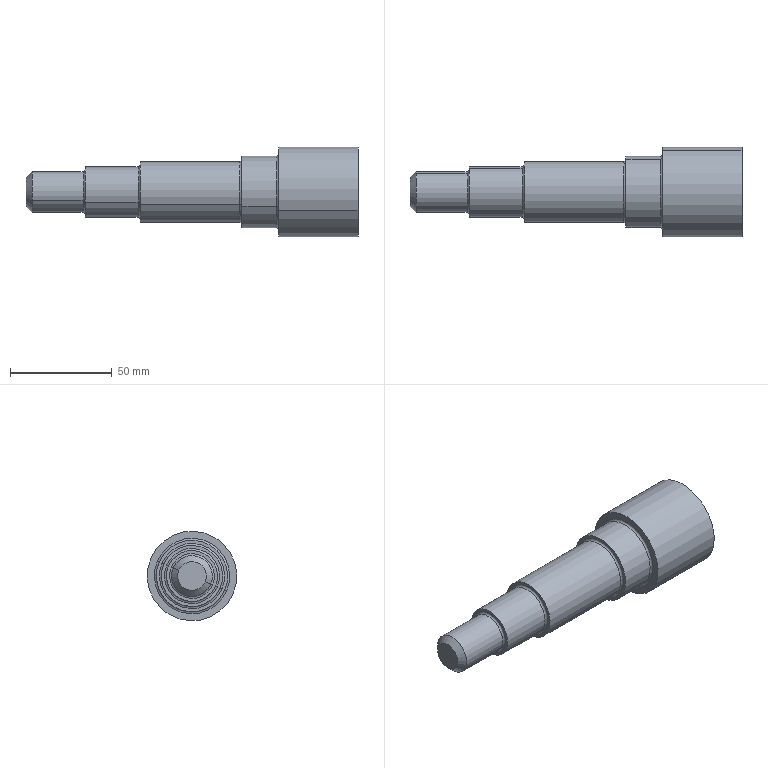Component | SolidWorks | AxisThree-1 | 1 solid | 26 faces | box 163 x 44 x 44 mm | volume 134147 mm3 | cylinder 10 | torus 8 | plane 6 | cone 2 | commonest cylinder face diameters 20 x2 25 x2 30 x2 35 x2 44 x2
build123d program:
from build123d import *


with BuildPart() as part:
    # Sketch1 → Revolve1 (revolve)
    with BuildSketch(Plane(origin=(0, 0, 0), x_dir=(0, 0, -1), z_dir=(1, 0, 0)), mode=Mode.PRIVATE) as revolve1_sk:
        with BuildLine():
            Line((0, 0), (0, 22))
            Line((0, 22), (39, 22))
            Line((39, 22), (39, 18.5))
            ThreePointArc((39, 18.5), (39.293, 17.793), (40, 17.5))
            Line((40, 17.5), (57, 17.5))
            Line((57, 17.5), (57, 16))
            ThreePointArc((57, 16), (57.293, 15.293), (58, 15))
            Line((58, 15), (107, 15))
            Line((107, 15), (107, 13.5))
            ThreePointArc((107, 13.5), (107.293, 12.793), (108, 12.5))
            Line((108, 12.5), (134, 12.5))
            Line((134, 12.5), (134, 11))
            ThreePointArc((134, 11), (134.293, 10.293), (135, 10))
            Line((135, 10), (160, 10))
            Line((160, 10), (163, 7))
            Line((163, 7), (163, 0))
            Line((163, 0), (0, 0))
        make_face()
    revolve(revolve1_sk.sketch.rotate(Axis((0, 0, -163), (0, 0, 1)), 90), axis=Axis((0, 0, -163), (0, 0, 1)))


solid = part.part

# Placed as in the assembly
solid = solid.moved(Location((528.528, 15.31, -240), (0, 90, 0)))
STEP:
#1=COLOUR_RGB('',0.7922,0.8196,0.9333);
#2=FILL_AREA_STYLE_COLOUR('',#1);
#3=FILL_AREA_STYLE('',(#2));
#4=SURFACE_STYLE_FILL_AREA(#3);
#5=SURFACE_SIDE_STYLE('',(#4));
#6=SURFACE_STYLE_USAGE(.BOTH.,#5);
#7=PRESENTATION_STYLE_ASSIGNMENT((#6));
#8=CARTESIAN_POINT('',(14.391,0.8549,-9.337));
#9=VERTEX_POINT('',#8);
#10=CARTESIAN_POINT('',(14.391,0.3507,-9.56));
#11=VERTEX_POINT('',#10);
#12=CARTESIAN_POINT('',(14.391,0.6028,-9.449));
#13=DIRECTION('',(-1.,0.,0.));
#14=DIRECTION('',(0.,0.9147,0.4041));
#15=AXIS2_PLACEMENT_3D('',#12,#13,#14);
#16=CIRCLE('',#15,0.2756);
#17=EDGE_CURVE('',#9,#11,#16,.T.);
#18=ORIENTED_EDGE('',*,*,#17,.F.);
#19=CARTESIAN_POINT('',(14.509,0.9629,-9.29));
#20=VERTEX_POINT('',#19);
#21=CARTESIAN_POINT('',(14.391,0.8549,-9.337));
#22=DIRECTION('',(0.7071,0.6468,0.2858));
#23=VECTOR('',#22,39.37);
#24=LINE('',#21,#23);
#25=EDGE_CURVE('',#9,#20,#24,.T.);
#26=ORIENTED_EDGE('',*,*,#25,.T.);
#27=CARTESIAN_POINT('',(14.509,0.2426,-9.608));
#28=VERTEX_POINT('',#27);
#29=CARTESIAN_POINT('',(14.509,0.6028,-9.449));
#30=DIRECTION('',(-1.,0.,0.));
#31=DIRECTION('',(0.,0.9147,0.4041));
#32=AXIS2_PLACEMENT_3D('',#29,#30,#31);
#33=CIRCLE('',#32,0.3937);
#34=EDGE_CURVE('',#20,#28,#33,.T.);
#35=ORIENTED_EDGE('',*,*,#34,.T.);
#36=CARTESIAN_POINT('',(14.391,0.3507,-9.56));
#37=DIRECTION('',(0.7071,-0.6468,-0.2858));
#38=VECTOR('',#37,39.37);
#39=LINE('',#36,#38);
#40=EDGE_CURVE('',#11,#28,#39,.T.);
#41=ORIENTED_EDGE('',*,*,#40,.F.);
#42=EDGE_LOOP('',(#18,#26,#35,#41));
#43=FACE_OUTER_BOUND('',#42,.T.);
#44=CARTESIAN_POINT('',(14.391,0.6028,-9.449));
#45=DIRECTION('',(1.,0.,0.));
#46=DIRECTION('',(0.,-0.9147,-0.4041));
#47=AXIS2_PLACEMENT_3D('',#44,#45,#46);
#48=CONICAL_SURFACE('',#47,0.2756,0.7854);
#49=ADVANCED_FACE('',(#43),#48,.T.);
#50=CARTESIAN_POINT('',(15.493,0.9629,-9.29));
#51=VERTEX_POINT('',#50);
#52=CARTESIAN_POINT('',(15.493,0.2426,-9.608));
#53=VERTEX_POINT('',#52);
#54=CARTESIAN_POINT('',(15.493,0.6028,-9.449));
#55=DIRECTION('',(-1.,0.,0.));
#56=DIRECTION('',(0.,0.9147,0.4041));
#57=AXIS2_PLACEMENT_3D('',#54,#55,#56);
#58=CIRCLE('',#57,0.3937);
#59=EDGE_CURVE('',#51,#53,#58,.T.);
#60=ORIENTED_EDGE('',*,*,#59,.T.);
#61=CARTESIAN_POINT('',(14.391,0.2426,-9.608));
#62=DIRECTION('',(-1.,0.,0.));
#63=VECTOR('',#62,39.37);
#64=LINE('',#61,#63);
#65=EDGE_CURVE('',#53,#28,#64,.T.);
#66=ORIENTED_EDGE('',*,*,#65,.T.);
#67=ORIENTED_EDGE('',*,*,#34,.F.);
#68=CARTESIAN_POINT('',(14.391,0.9629,-9.29));
#69=DIRECTION('',(-1.,0.,0.));
#70=VECTOR('',#69,39.37);
#71=LINE('',#68,#70);
#72=EDGE_CURVE('',#51,#20,#71,.T.);
#73=ORIENTED_EDGE('',*,*,#72,.F.);
#74=EDGE_LOOP('',(#60,#66,#67,#73));
#75=FACE_OUTER_BOUND('',#74,.T.);
#76=CARTESIAN_POINT('',(14.391,0.6028,-9.449));
#77=DIRECTION('',(-1.,0.,0.));
#78=DIRECTION('',(0.,0.9147,0.4041));
#79=AXIS2_PLACEMENT_3D('',#76,#77,#78);
#80=CYLINDRICAL_SURFACE('',#79,0.3937);
#81=ADVANCED_FACE('',(#75),#80,.T.);
#82=CARTESIAN_POINT('',(15.493,0.6028,-9.449));
#83=DIRECTION('',(-1.,0.,0.));
#84=DIRECTION('',(0.,0.9147,0.4041));
#85=AXIS2_PLACEMENT_3D('',#82,#83,#84);
#86=CIRCLE('',#85,0.3937);
#87=EDGE_CURVE('',#53,#51,#86,.T.);
#88=ORIENTED_EDGE('',*,*,#87,.F.);
#89=CARTESIAN_POINT('',(15.533,0.2066,-9.624));
#90=VERTEX_POINT('',#89);
#91=CARTESIAN_POINT('',(15.493,0.2066,-9.624));
#92=DIRECTION('',(0.,0.4041,-0.9147));
#93=DIRECTION('',(0.,0.9147,0.4041));
#94=AXIS2_PLACEMENT_3D('',#91,#92,#93);
#95=CIRCLE('',#94,0.03937);
#96=EDGE_CURVE('',#53,#90,#95,.T.);
#97=ORIENTED_EDGE('',*,*,#96,.T.);
#98=CARTESIAN_POINT('',(15.533,0.9989,-9.274));
#99=VERTEX_POINT('',#98);
#100=CARTESIAN_POINT('',(15.533,0.6028,-9.449));
#101=DIRECTION('',(-1.,0.,0.));
#102=DIRECTION('',(0.,0.9147,0.4041));
#103=AXIS2_PLACEMENT_3D('',#100,#101,#102);
#104=CIRCLE('',#103,0.4331);
#105=EDGE_CURVE('',#90,#99,#104,.T.);
#106=ORIENTED_EDGE('',*,*,#105,.T.);
#107=CARTESIAN_POINT('',(15.493,0.9989,-9.274));
#108=DIRECTION('',(0.,-0.4041,0.9147));
#109=DIRECTION('',(0.,-0.9147,-0.4041));
#110=AXIS2_PLACEMENT_3D('',#107,#108,#109);
#111=CIRCLE('',#110,0.03937);
#112=EDGE_CURVE('',#51,#99,#111,.T.);
#113=ORIENTED_EDGE('',*,*,#112,.F.);
#114=EDGE_LOOP('',(#88,#97,#106,#113));
#115=FACE_OUTER_BOUND('',#114,.T.);
#116=CARTESIAN_POINT('',(15.493,0.6028,-9.449));
#117=DIRECTION('',(-1.,0.,0.));
#118=DIRECTION('',(0.,0.9147,0.4041));
#119=AXIS2_PLACEMENT_3D('',#116,#117,#118);
#120=TOROIDAL_SURFACE('',#119,0.4331,0.03937);
#121=ADVANCED_FACE('',(#115),#120,.F.);
#122=CARTESIAN_POINT('',(16.556,1.053,-9.25));
#123=VERTEX_POINT('',#122);
#124=CARTESIAN_POINT('',(16.556,0.1526,-9.648));
#125=VERTEX_POINT('',#124);
#126=CARTESIAN_POINT('',(16.556,0.6028,-9.449));
#127=DIRECTION('',(-1.,0.,0.));
#128=DIRECTION('',(0.,0.9147,0.4041));
#129=AXIS2_PLACEMENT_3D('',#126,#127,#128);
#130=CIRCLE('',#129,0.4921);
#131=EDGE_CURVE('',#123,#125,#130,.T.);
#132=ORIENTED_EDGE('',*,*,#131,.T.);
#133=CARTESIAN_POINT('',(15.533,0.1526,-9.648));
#134=VERTEX_POINT('',#133);
#135=CARTESIAN_POINT('',(14.391,0.1526,-9.648));
#136=DIRECTION('',(-1.,0.,0.));
#137=VECTOR('',#136,39.37);
#138=LINE('',#135,#137);
#139=EDGE_CURVE('',#125,#134,#138,.T.);
#140=ORIENTED_EDGE('',*,*,#139,.T.);
#141=CARTESIAN_POINT('',(15.533,1.053,-9.25));
#142=VERTEX_POINT('',#141);
#143=CARTESIAN_POINT('',(15.533,0.6028,-9.449));
#144=DIRECTION('',(-1.,0.,0.));
#145=DIRECTION('',(0.,0.9147,0.4041));
#146=AXIS2_PLACEMENT_3D('',#143,#144,#145);
#147=CIRCLE('',#146,0.4921);
#148=EDGE_CURVE('',#142,#134,#147,.T.);
#149=ORIENTED_EDGE('',*,*,#148,.F.);
#150=CARTESIAN_POINT('',(14.391,1.053,-9.25));
#151=DIRECTION('',(-1.,0.,0.));
#152=VECTOR('',#151,39.37);
#153=LINE('',#150,#152);
#154=EDGE_CURVE('',#123,#142,#153,.T.);
#155=ORIENTED_EDGE('',*,*,#154,.F.);
#156=EDGE_LOOP('',(#132,#140,#149,#155));
#157=FACE_OUTER_BOUND('',#156,.T.);
#158=CARTESIAN_POINT('',(14.391,0.6028,-9.449));
#159=DIRECTION('',(-1.,0.,0.));
#160=DIRECTION('',(0.,0.9147,0.4041));
#161=AXIS2_PLACEMENT_3D('',#158,#159,#160);
#162=CYLINDRICAL_SURFACE('',#161,0.4921);
#163=ADVANCED_FACE('',(#157),#162,.T.);
#164=CARTESIAN_POINT('',(16.556,0.6028,-9.449));
#165=DIRECTION('',(-1.,0.,0.));
#166=DIRECTION('',(0.,0.9147,0.4041));
#167=AXIS2_PLACEMENT_3D('',#164,#165,#166);
#168=CIRCLE('',#167,0.4921);
#169=EDGE_CURVE('',#125,#123,#168,.T.);
#170=ORIENTED_EDGE('',*,*,#169,.F.);
#171=CARTESIAN_POINT('',(16.596,0.1166,-9.664));
#172=VERTEX_POINT('',#171);
#173=CARTESIAN_POINT('',(16.556,0.1166,-9.664));
#174=DIRECTION('',(0.,0.4041,-0.9147));
#175=DIRECTION('',(0.,0.9147,0.4041));
#176=AXIS2_PLACEMENT_3D('',#173,#174,#175);
#177=CIRCLE('',#176,0.03937);
#178=EDGE_CURVE('',#125,#172,#177,.T.);
#179=ORIENTED_EDGE('',*,*,#178,.T.);
#180=CARTESIAN_POINT('',(16.596,1.089,-9.234));
#181=VERTEX_POINT('',#180);
#182=CARTESIAN_POINT('',(16.596,0.6028,-9.449));
#183=DIRECTION('',(-1.,0.,0.));
#184=DIRECTION('',(0.,0.9147,0.4041));
#185=AXIS2_PLACEMENT_3D('',#182,#183,#184);
#186=CIRCLE('',#185,0.5315);
#187=EDGE_CURVE('',#172,#181,#186,.T.);
#188=ORIENTED_EDGE('',*,*,#187,.T.);
#189=CARTESIAN_POINT('',(16.556,1.089,-9.234));
#190=DIRECTION('',(0.,-0.4041,0.9147));
#191=DIRECTION('',(0.,-0.9147,-0.4041));
#192=AXIS2_PLACEMENT_3D('',#189,#190,#191);
#193=CIRCLE('',#192,0.03937);
#194=EDGE_CURVE('',#123,#181,#193,.T.);
#195=ORIENTED_EDGE('',*,*,#194,.F.);
#196=EDGE_LOOP('',(#170,#179,#188,#195));
#197=FACE_OUTER_BOUND('',#196,.T.);
#198=CARTESIAN_POINT('',(16.556,0.6028,-9.449));
#199=DIRECTION('',(-1.,0.,0.));
#200=DIRECTION('',(0.,0.9147,0.4041));
#201=AXIS2_PLACEMENT_3D('',#198,#199,#200);
#202=TOROIDAL_SURFACE('',#201,0.5315,0.03937);
#203=ADVANCED_FACE('',(#197),#202,.F.);
#204=CARTESIAN_POINT('',(18.525,1.143,-9.21));
#205=VERTEX_POINT('',#204);
#206=CARTESIAN_POINT('',(18.525,0.06259,-9.687));
#207=VERTEX_POINT('',#206);
#208=CARTESIAN_POINT('',(18.525,0.6028,-9.449));
#209=DIRECTION('',(-1.,0.,0.));
#210=DIRECTION('',(0.,0.9147,0.4041));
#211=AXIS2_PLACEMENT_3D('',#208,#209,#210);
#212=CIRCLE('',#211,0.5906);
#213=EDGE_CURVE('',#205,#207,#212,.T.);
#214=ORIENTED_EDGE('',*,*,#213,.T.);
#215=CARTESIAN_POINT('',(16.596,0.06259,-9.687));
#216=VERTEX_POINT('',#215);
#217=CARTESIAN_POINT('',(14.391,0.06259,-9.687));
#218=DIRECTION('',(-1.,0.,0.));
#219=VECTOR('',#218,39.37);
#220=LINE('',#217,#219);
#221=EDGE_CURVE('',#207,#216,#220,.T.);
#222=ORIENTED_EDGE('',*,*,#221,.T.);
#223=CARTESIAN_POINT('',(16.596,1.143,-9.21));
#224=VERTEX_POINT('',#223);
#225=CARTESIAN_POINT('',(16.596,0.6028,-9.449));
#226=DIRECTION('',(-1.,0.,0.));
#227=DIRECTION('',(0.,0.9147,0.4041));
#228=AXIS2_PLACEMENT_3D('',#225,#226,#227);
#229=CIRCLE('',#228,0.5906);
#230=EDGE_CURVE('',#224,#216,#229,.T.);
#231=ORIENTED_EDGE('',*,*,#230,.F.);
#232=CARTESIAN_POINT('',(14.391,1.143,-9.21));
#233=DIRECTION('',(-1.,0.,0.));
#234=VECTOR('',#233,39.37);
#235=LINE('',#232,#234);
#236=EDGE_CURVE('',#205,#224,#235,.T.);
#237=ORIENTED_EDGE('',*,*,#236,.F.);
#238=EDGE_LOOP('',(#214,#222,#231,#237));
#239=FACE_OUTER_BOUND('',#238,.T.);
#240=CARTESIAN_POINT('',(14.391,0.6028,-9.449));
#241=DIRECTION('',(-1.,0.,0.));
#242=DIRECTION('',(0.,0.9147,0.4041));
#243=AXIS2_PLACEMENT_3D('',#240,#241,#242);
#244=CYLINDRICAL_SURFACE('',#243,0.5906);
#245=ADVANCED_FACE('',(#239),#244,.T.);
#246=CARTESIAN_POINT('',(18.525,0.6028,-9.449));
#247=DIRECTION('',(-1.,0.,0.));
#248=DIRECTION('',(0.,0.9147,0.4041));
#249=AXIS2_PLACEMENT_3D('',#246,#247,#248);
#250=CIRCLE('',#249,0.5906);
#251=EDGE_CURVE('',#207,#205,#250,.T.);
#252=ORIENTED_EDGE('',*,*,#251,.F.);
#253=CARTESIAN_POINT('',(18.564,0.02658,-9.703));
#254=VERTEX_POINT('',#253);
#255=CARTESIAN_POINT('',(18.525,0.02658,-9.703));
#256=DIRECTION('',(0.,0.4041,-0.9147));
#257=DIRECTION('',(0.,0.9147,0.4041));
#258=AXIS2_PLACEMENT_3D('',#255,#256,#257);
#259=CIRCLE('',#258,0.03937);
#260=EDGE_CURVE('',#207,#254,#259,.T.);
#261=ORIENTED_EDGE('',*,*,#260,.T.);
#262=CARTESIAN_POINT('',(18.564,1.179,-9.194));
#263=VERTEX_POINT('',#262);
#264=CARTESIAN_POINT('',(18.564,0.6028,-9.449));
#265=DIRECTION('',(-1.,0.,0.));
#266=DIRECTION('',(0.,0.9147,0.4041));
#267=AXIS2_PLACEMENT_3D('',#264,#265,#266);
#268=CIRCLE('',#267,0.6299);
#269=EDGE_CURVE('',#254,#263,#268,.T.);
#270=ORIENTED_EDGE('',*,*,#269,.T.);
#271=CARTESIAN_POINT('',(18.525,1.179,-9.194));
#272=DIRECTION('',(0.,-0.4041,0.9147));
#273=DIRECTION('',(0.,-0.9147,-0.4041));
#274=AXIS2_PLACEMENT_3D('',#271,#272,#273);
#275=CIRCLE('',#274,0.03937);
#276=EDGE_CURVE('',#205,#263,#275,.T.);
#277=ORIENTED_EDGE('',*,*,#276,.F.);
#278=EDGE_LOOP('',(#252,#261,#270,#277));
#279=FACE_OUTER_BOUND('',#278,.T.);
#280=CARTESIAN_POINT('',(18.525,0.6028,-9.449));
#281=DIRECTION('',(-1.,0.,0.));
#282=DIRECTION('',(0.,0.9147,0.4041));
#283=AXIS2_PLACEMENT_3D('',#280,#281,#282);
#284=TOROIDAL_SURFACE('',#283,0.6299,0.03937);
#285=ADVANCED_FACE('',(#279),#284,.F.);
#286=CARTESIAN_POINT('',(19.233,1.233,-9.17));
#287=VERTEX_POINT('',#286);
#288=CARTESIAN_POINT('',(19.233,-0.02744,-9.727));
#289=VERTEX_POINT('',#288);
#290=CARTESIAN_POINT('',(19.233,0.6028,-9.449));
#291=DIRECTION('',(-1.,0.,0.));
#292=DIRECTION('',(0.,0.9147,0.4041));
#293=AXIS2_PLACEMENT_3D('',#290,#291,#292);
#294=CIRCLE('',#293,0.689);
#295=EDGE_CURVE('',#287,#289,#294,.T.);
#296=ORIENTED_EDGE('',*,*,#295,.T.);
#297=CARTESIAN_POINT('',(18.564,-0.02744,-9.727));
#298=VERTEX_POINT('',#297);
#299=CARTESIAN_POINT('',(14.391,-0.02744,-9.727));
#300=DIRECTION('',(-1.,0.,0.));
#301=VECTOR('',#300,39.37);
#302=LINE('',#299,#301);
#303=EDGE_CURVE('',#289,#298,#302,.T.);
#304=ORIENTED_EDGE('',*,*,#303,.T.);
#305=CARTESIAN_POINT('',(18.564,1.233,-9.17));
#306=VERTEX_POINT('',#305);
#307=CARTESIAN_POINT('',(18.564,0.6028,-9.449));
#308=DIRECTION('',(-1.,0.,0.));
#309=DIRECTION('',(0.,0.9147,0.4041));
#310=AXIS2_PLACEMENT_3D('',#307,#308,#309);
#311=CIRCLE('',#310,0.689);
#312=EDGE_CURVE('',#306,#298,#311,.T.);
#313=ORIENTED_EDGE('',*,*,#312,.F.);
#314=CARTESIAN_POINT('',(14.391,1.233,-9.17));
#315=DIRECTION('',(-1.,0.,0.));
#316=VECTOR('',#315,39.37);
#317=LINE('',#314,#316);
#318=EDGE_CURVE('',#287,#306,#317,.T.);
#319=ORIENTED_EDGE('',*,*,#318,.F.);
#320=EDGE_LOOP('',(#296,#304,#313,#319));
#321=FACE_OUTER_BOUND('',#320,.T.);
#322=CARTESIAN_POINT('',(14.391,0.6028,-9.449));
#323=DIRECTION('',(-1.,0.,0.));
#324=DIRECTION('',(0.,0.9147,0.4041));
#325=AXIS2_PLACEMENT_3D('',#322,#323,#324);
#326=CYLINDRICAL_SURFACE('',#325,0.689);
#327=ADVANCED_FACE('',(#321),#326,.T.);
#328=CARTESIAN_POINT('',(19.233,0.6028,-9.449));
#329=DIRECTION('',(-1.,0.,0.));
#330=DIRECTION('',(0.,0.9147,0.4041));
#331=AXIS2_PLACEMENT_3D('',#328,#329,#330);
#332=CIRCLE('',#331,0.689);
#333=EDGE_CURVE('',#289,#287,#332,.T.);
#334=ORIENTED_EDGE('',*,*,#333,.F.);
#335=CARTESIAN_POINT('',(19.273,-0.06345,-9.743));
#336=VERTEX_POINT('',#335);
#337=CARTESIAN_POINT('',(19.233,-0.06345,-9.743));
#338=DIRECTION('',(0.,0.4041,-0.9147));
#339=DIRECTION('',(0.,0.9147,0.4041));
#340=AXIS2_PLACEMENT_3D('',#337,#338,#339);
#341=CIRCLE('',#340,0.03937);
#342=EDGE_CURVE('',#289,#336,#341,.T.);
#343=ORIENTED_EDGE('',*,*,#342,.T.);
#344=CARTESIAN_POINT('',(19.273,1.269,-9.154));
#345=VERTEX_POINT('',#344);
#346=CARTESIAN_POINT('',(19.273,0.6028,-9.449));
#347=DIRECTION('',(-1.,0.,0.));
#348=DIRECTION('',(0.,0.9147,0.4041));
#349=AXIS2_PLACEMENT_3D('',#346,#347,#348);
#350=CIRCLE('',#349,0.7283);
#351=EDGE_CURVE('',#336,#345,#350,.T.);
#352=ORIENTED_EDGE('',*,*,#351,.T.);
#353=CARTESIAN_POINT('',(19.233,1.269,-9.154));
#354=DIRECTION('',(0.,-0.4041,0.9147));
#355=DIRECTION('',(0.,-0.9147,-0.4041));
#356=AXIS2_PLACEMENT_3D('',#353,#354,#355);
#357=CIRCLE('',#356,0.03937);
#358=EDGE_CURVE('',#287,#345,#357,.T.);
#359=ORIENTED_EDGE('',*,*,#358,.F.);
#360=EDGE_LOOP('',(#334,#343,#352,#359));
#361=FACE_OUTER_BOUND('',#360,.T.);
#362=CARTESIAN_POINT('',(19.233,0.6028,-9.449));
#363=DIRECTION('',(-1.,0.,0.));
#364=DIRECTION('',(0.,0.9147,0.4041));
#365=AXIS2_PLACEMENT_3D('',#362,#363,#364);
#366=TOROIDAL_SURFACE('',#365,0.7283,0.03937);
#367=ADVANCED_FACE('',(#361),#366,.F.);
#368=CARTESIAN_POINT('',(20.808,1.395,-9.099));
#369=VERTEX_POINT('',#368);
#370=CARTESIAN_POINT('',(20.808,-0.1895,-9.799));
#371=VERTEX_POINT('',#370);
#372=CARTESIAN_POINT('',(20.808,0.6028,-9.449));
#373=DIRECTION('',(-1.,0.,0.));
#374=DIRECTION('',(0.,0.9147,0.4041));
#375=AXIS2_PLACEMENT_3D('',#372,#373,#374);
#376=CIRCLE('',#375,0.8661);
#377=EDGE_CURVE('',#369,#371,#376,.T.);
#378=ORIENTED_EDGE('',*,*,#377,.T.);
#379=CARTESIAN_POINT('',(19.273,-0.1895,-9.799));
#380=VERTEX_POINT('',#379);
#381=CARTESIAN_POINT('',(14.391,-0.1895,-9.799));
#382=DIRECTION('',(-1.,0.,0.));
#383=VECTOR('',#382,39.37);
#384=LINE('',#381,#383);
#385=EDGE_CURVE('',#371,#380,#384,.T.);
#386=ORIENTED_EDGE('',*,*,#385,.T.);
#387=CARTESIAN_POINT('',(19.273,1.395,-9.099));
#388=VERTEX_POINT('',#387);
#389=CARTESIAN_POINT('',(19.273,0.6028,-9.449));
#390=DIRECTION('',(-1.,0.,0.));
#391=DIRECTION('',(0.,0.9147,0.4041));
#392=AXIS2_PLACEMENT_3D('',#389,#390,#391);
#393=CIRCLE('',#392,0.8661);
#394=EDGE_CURVE('',#388,#380,#393,.T.);
#395=ORIENTED_EDGE('',*,*,#394,.F.);
#396=CARTESIAN_POINT('',(14.391,1.395,-9.099));
#397=DIRECTION('',(-1.,0.,0.));
#398=VECTOR('',#397,39.37);
#399=LINE('',#396,#398);
#400=EDGE_CURVE('',#369,#388,#399,.T.);
#401=ORIENTED_EDGE('',*,*,#400,.F.);
#402=EDGE_LOOP('',(#378,#386,#395,#401));
#403=FACE_OUTER_BOUND('',#402,.T.);
#404=CARTESIAN_POINT('',(14.391,0.6028,-9.449));
#405=DIRECTION('',(-1.,0.,0.));
#406=DIRECTION('',(0.,0.9147,0.4041));
#407=AXIS2_PLACEMENT_3D('',#404,#405,#406);
#408=CYLINDRICAL_SURFACE('',#407,0.8661);
#409=ADVANCED_FACE('',(#403),#408,.T.);
#410=ORIENTED_EDGE('',*,*,#377,.F.);
#411=CARTESIAN_POINT('',(20.808,0.6028,-9.449));
#412=DIRECTION('',(-1.,0.,0.));
#413=DIRECTION('',(0.,0.9147,0.4041));
#414=AXIS2_PLACEMENT_3D('',#411,#412,#413);
#415=CIRCLE('',#414,0.8661);
#416=EDGE_CURVE('',#371,#369,#415,.T.);
#417=ORIENTED_EDGE('',*,*,#416,.F.);
#418=EDGE_LOOP('',(#410,#417));
#419=FACE_OUTER_BOUND('',#418,.T.);
#420=CARTESIAN_POINT('',(20.808,0.6028,-9.449));
#421=DIRECTION('',(1.,0.,0.));
#422=DIRECTION('',(0.,-0.9147,-0.4041));
#423=AXIS2_PLACEMENT_3D('',#420,#421,#422);
#424=PLANE('',#423);
#425=ADVANCED_FACE('',(#419),#424,.T.);
#426=ORIENTED_EDGE('',*,*,#385,.F.);
#427=ORIENTED_EDGE('',*,*,#416,.T.);
#428=ORIENTED_EDGE('',*,*,#400,.T.);
#429=CARTESIAN_POINT('',(19.273,0.6028,-9.449));
#430=DIRECTION('',(-1.,0.,0.));
#431=DIRECTION('',(0.,0.9147,0.4041));
#432=AXIS2_PLACEMENT_3D('',#429,#430,#431);
#433=CIRCLE('',#432,0.8661);
#434=EDGE_CURVE('',#380,#388,#433,.T.);
#435=ORIENTED_EDGE('',*,*,#434,.F.);
#436=EDGE_LOOP('',(#426,#427,#428,#435));
#437=FACE_OUTER_BOUND('',#436,.T.);
#438=CARTESIAN_POINT('',(14.391,0.6028,-9.449));
#439=DIRECTION('',(-1.,0.,0.));
#440=DIRECTION('',(0.,0.9147,0.4041));
#441=AXIS2_PLACEMENT_3D('',#438,#439,#440);
#442=CYLINDRICAL_SURFACE('',#441,0.8661);
#443=ADVANCED_FACE('',(#437),#442,.T.);
#444=ORIENTED_EDGE('',*,*,#394,.T.);
#445=ORIENTED_EDGE('',*,*,#434,.T.);
#446=EDGE_LOOP('',(#444,#445));
#447=FACE_OUTER_BOUND('',#446,.T.);
#448=CARTESIAN_POINT('',(19.273,0.6028,-9.449));
#449=DIRECTION('',(-1.,0.,0.));
#450=DIRECTION('',(0.,0.9147,0.4041));
#451=AXIS2_PLACEMENT_3D('',#448,#449,#450);
#452=CIRCLE('',#451,0.7283);
#453=EDGE_CURVE('',#345,#336,#452,.T.);
#454=ORIENTED_EDGE('',*,*,#453,.F.);
#455=ORIENTED_EDGE('',*,*,#351,.F.);
#456=EDGE_LOOP('',(#454,#455));
#457=FACE_BOUND('',#456,.T.);
#458=CARTESIAN_POINT('',(19.273,0.9528,-10.241));
#459=DIRECTION('',(-1.,0.,0.));
#460=DIRECTION('',(0.,0.9147,0.4041));
#461=AXIS2_PLACEMENT_3D('',#458,#459,#460);
#462=PLANE('',#461);
#463=ADVANCED_FACE('',(#447,#457),#462,.T.);
#464=ORIENTED_EDGE('',*,*,#342,.F.);
#465=ORIENTED_EDGE('',*,*,#295,.F.);
#466=ORIENTED_EDGE('',*,*,#358,.T.);
#467=ORIENTED_EDGE('',*,*,#453,.T.);
#468=EDGE_LOOP('',(#464,#465,#466,#467));
#469=FACE_OUTER_BOUND('',#468,.T.);
#470=CARTESIAN_POINT('',(19.233,0.6028,-9.449));
#471=DIRECTION('',(-1.,0.,0.));
#472=DIRECTION('',(0.,0.9147,0.4041));
#473=AXIS2_PLACEMENT_3D('',#470,#471,#472);
#474=TOROIDAL_SURFACE('',#473,0.7283,0.03937);
#475=ADVANCED_FACE('',(#469),#474,.F.);
#476=ORIENTED_EDGE('',*,*,#303,.F.);
#477=ORIENTED_EDGE('',*,*,#333,.T.);
#478=ORIENTED_EDGE('',*,*,#318,.T.);
#479=CARTESIAN_POINT('',(18.564,0.6028,-9.449));
#480=DIRECTION('',(-1.,0.,0.));
#481=DIRECTION('',(0.,0.9147,0.4041));
#482=AXIS2_PLACEMENT_3D('',#479,#480,#481);
#483=CIRCLE('',#482,0.689);
#484=EDGE_CURVE('',#298,#306,#483,.T.);
#485=ORIENTED_EDGE('',*,*,#484,.F.);
#486=EDGE_LOOP('',(#476,#477,#478,#485));
#487=FACE_OUTER_BOUND('',#486,.T.);
#488=CARTESIAN_POINT('',(14.391,0.6028,-9.449));
#489=DIRECTION('',(-1.,0.,0.));
#490=DIRECTION('',(0.,0.9147,0.4041));
#491=AXIS2_PLACEMENT_3D('',#488,#489,#490);
#492=CYLINDRICAL_SURFACE('',#491,0.689);
#493=ADVANCED_FACE('',(#487),#492,.T.);
#494=ORIENTED_EDGE('',*,*,#312,.T.);
#495=ORIENTED_EDGE('',*,*,#484,.T.);
#496=EDGE_LOOP('',(#494,#495));
#497=FACE_OUTER_BOUND('',#496,.T.);
#498=CARTESIAN_POINT('',(18.564,0.6028,-9.449));
#499=DIRECTION('',(-1.,0.,0.));
#500=DIRECTION('',(0.,0.9147,0.4041));
#501=AXIS2_PLACEMENT_3D('',#498,#499,#500);
#502=CIRCLE('',#501,0.6299);
#503=EDGE_CURVE('',#263,#254,#502,.T.);
#504=ORIENTED_EDGE('',*,*,#503,.F.);
#505=ORIENTED_EDGE('',*,*,#269,.F.);
#506=EDGE_LOOP('',(#504,#505));
#507=FACE_BOUND('',#506,.T.);
#508=CARTESIAN_POINT('',(18.564,0.8812,-10.079));
#509=DIRECTION('',(-1.,0.,0.));
#510=DIRECTION('',(0.,0.9147,0.4041));
#511=AXIS2_PLACEMENT_3D('',#508,#509,#510);
#512=PLANE('',#511);
#513=ADVANCED_FACE('',(#497,#507),#512,.T.);
#514=ORIENTED_EDGE('',*,*,#260,.F.);
#515=ORIENTED_EDGE('',*,*,#213,.F.);
#516=ORIENTED_EDGE('',*,*,#276,.T.);
#517=ORIENTED_EDGE('',*,*,#503,.T.);
#518=EDGE_LOOP('',(#514,#515,#516,#517));
#519=FACE_OUTER_BOUND('',#518,.T.);
#520=CARTESIAN_POINT('',(18.525,0.6028,-9.449));
#521=DIRECTION('',(-1.,0.,0.));
#522=DIRECTION('',(0.,0.9147,0.4041));
#523=AXIS2_PLACEMENT_3D('',#520,#521,#522);
#524=TOROIDAL_SURFACE('',#523,0.6299,0.03937);
#525=ADVANCED_FACE('',(#519),#524,.F.);
#526=ORIENTED_EDGE('',*,*,#221,.F.);
#527=ORIENTED_EDGE('',*,*,#251,.T.);
#528=ORIENTED_EDGE('',*,*,#236,.T.);
#529=CARTESIAN_POINT('',(16.596,0.6028,-9.449));
#530=DIRECTION('',(-1.,0.,0.));
#531=DIRECTION('',(0.,0.9147,0.4041));
#532=AXIS2_PLACEMENT_3D('',#529,#530,#531);
#533=CIRCLE('',#532,0.5906);
#534=EDGE_CURVE('',#216,#224,#533,.T.);
#535=ORIENTED_EDGE('',*,*,#534,.F.);
#536=EDGE_LOOP('',(#526,#527,#528,#535));
#537=FACE_OUTER_BOUND('',#536,.T.);
#538=CARTESIAN_POINT('',(14.391,0.6028,-9.449));
#539=DIRECTION('',(-1.,0.,0.));
#540=DIRECTION('',(0.,0.9147,0.4041));
#541=AXIS2_PLACEMENT_3D('',#538,#539,#540);
#542=CYLINDRICAL_SURFACE('',#541,0.5906);
#543=ADVANCED_FACE('',(#537),#542,.T.);
#544=ORIENTED_EDGE('',*,*,#230,.T.);
#545=ORIENTED_EDGE('',*,*,#534,.T.);
#546=EDGE_LOOP('',(#544,#545));
#547=FACE_OUTER_BOUND('',#546,.T.);
#548=CARTESIAN_POINT('',(16.596,0.6028,-9.449));
#549=DIRECTION('',(-1.,0.,0.));
#550=DIRECTION('',(0.,0.9147,0.4041));
#551=AXIS2_PLACEMENT_3D('',#548,#549,#550);
#552=CIRCLE('',#551,0.5315);
#553=EDGE_CURVE('',#181,#172,#552,.T.);
#554=ORIENTED_EDGE('',*,*,#553,.F.);
#555=ORIENTED_EDGE('',*,*,#187,.F.);
#556=EDGE_LOOP('',(#554,#555));
#557=FACE_BOUND('',#556,.T.);
#558=CARTESIAN_POINT('',(16.596,0.8414,-9.989));
#559=DIRECTION('',(-1.,0.,0.));
#560=DIRECTION('',(0.,0.9147,0.4041));
#561=AXIS2_PLACEMENT_3D('',#558,#559,#560);
#562=PLANE('',#561);
#563=ADVANCED_FACE('',(#547,#557),#562,.T.);
#564=ORIENTED_EDGE('',*,*,#178,.F.);
#565=ORIENTED_EDGE('',*,*,#131,.F.);
#566=ORIENTED_EDGE('',*,*,#194,.T.);
#567=ORIENTED_EDGE('',*,*,#553,.T.);
#568=EDGE_LOOP('',(#564,#565,#566,#567));
#569=FACE_OUTER_BOUND('',#568,.T.);
#570=CARTESIAN_POINT('',(16.556,0.6028,-9.449));
#571=DIRECTION('',(-1.,0.,0.));
#572=DIRECTION('',(0.,0.9147,0.4041));
#573=AXIS2_PLACEMENT_3D('',#570,#571,#572);
#574=TOROIDAL_SURFACE('',#573,0.5315,0.03937);
#575=ADVANCED_FACE('',(#569),#574,.F.);
#576=ORIENTED_EDGE('',*,*,#139,.F.);
#577=ORIENTED_EDGE('',*,*,#169,.T.);
#578=ORIENTED_EDGE('',*,*,#154,.T.);
#579=CARTESIAN_POINT('',(15.533,0.6028,-9.449));
#580=DIRECTION('',(-1.,0.,0.));
#581=DIRECTION('',(0.,0.9147,0.4041));
#582=AXIS2_PLACEMENT_3D('',#579,#580,#581);
#583=CIRCLE('',#582,0.4921);
#584=EDGE_CURVE('',#134,#142,#583,.T.);
#585=ORIENTED_EDGE('',*,*,#584,.F.);
#586=EDGE_LOOP('',(#576,#577,#578,#585));
#587=FACE_OUTER_BOUND('',#586,.T.);
#588=CARTESIAN_POINT('',(14.391,0.6028,-9.449));
#589=DIRECTION('',(-1.,0.,0.));
#590=DIRECTION('',(0.,0.9147,0.4041));
#591=AXIS2_PLACEMENT_3D('',#588,#589,#590);
#592=CYLINDRICAL_SURFACE('',#591,0.4921);
#593=ADVANCED_FACE('',(#587),#592,.T.);
#594=ORIENTED_EDGE('',*,*,#148,.T.);
#595=ORIENTED_EDGE('',*,*,#584,.T.);
#596=EDGE_LOOP('',(#594,#595));
#597=FACE_OUTER_BOUND('',#596,.T.);
#598=CARTESIAN_POINT('',(15.533,0.6028,-9.449));
#599=DIRECTION('',(-1.,0.,0.));
#600=DIRECTION('',(0.,0.9147,0.4041));
#601=AXIS2_PLACEMENT_3D('',#598,#599,#600);
#602=CIRCLE('',#601,0.4331);
#603=EDGE_CURVE('',#99,#90,#602,.T.);
#604=ORIENTED_EDGE('',*,*,#603,.F.);
#605=ORIENTED_EDGE('',*,*,#105,.F.);
#606=EDGE_LOOP('',(#604,#605));
#607=FACE_BOUND('',#606,.T.);
#608=CARTESIAN_POINT('',(15.533,0.8016,-9.899));
#609=DIRECTION('',(-1.,0.,0.));
#610=DIRECTION('',(0.,0.9147,0.4041));
#611=AXIS2_PLACEMENT_3D('',#608,#609,#610);
#612=PLANE('',#611);
#613=ADVANCED_FACE('',(#597,#607),#612,.T.);
#614=ORIENTED_EDGE('',*,*,#96,.F.);
#615=ORIENTED_EDGE('',*,*,#59,.F.);
#616=ORIENTED_EDGE('',*,*,#112,.T.);
#617=ORIENTED_EDGE('',*,*,#603,.T.);
#618=EDGE_LOOP('',(#614,#615,#616,#617));
#619=FACE_OUTER_BOUND('',#618,.T.);
#620=CARTESIAN_POINT('',(15.493,0.6028,-9.449));
#621=DIRECTION('',(-1.,0.,0.));
#622=DIRECTION('',(0.,0.9147,0.4041));
#623=AXIS2_PLACEMENT_3D('',#620,#621,#622);
#624=TOROIDAL_SURFACE('',#623,0.4331,0.03937);
#625=ADVANCED_FACE('',(#619),#624,.F.);
#626=ORIENTED_EDGE('',*,*,#65,.F.);
#627=ORIENTED_EDGE('',*,*,#87,.T.);
#628=ORIENTED_EDGE('',*,*,#72,.T.);
#629=CARTESIAN_POINT('',(14.509,0.6028,-9.449));
#630=DIRECTION('',(-1.,0.,0.));
#631=DIRECTION('',(0.,0.9147,0.4041));
#632=AXIS2_PLACEMENT_3D('',#629,#630,#631);
#633=CIRCLE('',#632,0.3937);
#634=EDGE_CURVE('',#28,#20,#633,.T.);
#635=ORIENTED_EDGE('',*,*,#634,.F.);
#636=EDGE_LOOP('',(#626,#627,#628,#635));
#637=FACE_OUTER_BOUND('',#636,.T.);
#638=CARTESIAN_POINT('',(14.391,0.6028,-9.449));
#639=DIRECTION('',(-1.,0.,0.));
#640=DIRECTION('',(0.,0.9147,0.4041));
#641=AXIS2_PLACEMENT_3D('',#638,#639,#640);
#642=CYLINDRICAL_SURFACE('',#641,0.3937);
#643=ADVANCED_FACE('',(#637),#642,.T.);
#644=ORIENTED_EDGE('',*,*,#25,.F.);
#645=CARTESIAN_POINT('',(14.391,0.6028,-9.449));
#646=DIRECTION('',(-1.,0.,0.));
#647=DIRECTION('',(0.,0.9147,0.4041));
#648=AXIS2_PLACEMENT_3D('',#645,#646,#647);
#649=CIRCLE('',#648,0.2756);
#650=EDGE_CURVE('',#11,#9,#649,.T.);
#651=ORIENTED_EDGE('',*,*,#650,.F.);
#652=ORIENTED_EDGE('',*,*,#40,.T.);
#653=ORIENTED_EDGE('',*,*,#634,.T.);
#654=EDGE_LOOP('',(#644,#651,#652,#653));
#655=FACE_OUTER_BOUND('',#654,.T.);
#656=CARTESIAN_POINT('',(14.391,0.6028,-9.449));
#657=DIRECTION('',(1.,0.,0.));
#658=DIRECTION('',(0.,-0.9147,-0.4041));
#659=AXIS2_PLACEMENT_3D('',#656,#657,#658);
#660=CONICAL_SURFACE('',#659,0.2756,0.7854);
#661=ADVANCED_FACE('',(#655),#660,.T.);
#662=ORIENTED_EDGE('',*,*,#650,.T.);
#663=ORIENTED_EDGE('',*,*,#17,.T.);
#664=EDGE_LOOP('',(#662,#663));
#665=FACE_OUTER_BOUND('',#664,.T.);
#666=CARTESIAN_POINT('',(14.391,0.7141,-9.701));
#667=DIRECTION('',(-1.,0.,0.));
#668=DIRECTION('',(0.,0.9147,0.4041));
#669=AXIS2_PLACEMENT_3D('',#666,#667,#668);
#670=PLANE('',#669);
#671=ADVANCED_FACE('',(#665),#670,.T.);
#672=CLOSED_SHELL('',(#49,#81,#121,#163,#203,#245,#285,#327,#367,#409,#425,#443,#463,#475,#493,#513,#525,#543,#563,#575,#593,#613,#625,#643,#661,#671));
#673=MANIFOLD_SOLID_BREP('',#672);
#674=STYLED_ITEM('',(#7),#673);
#675=PRESENTATION_LAYER_ASSIGNMENT('','',(#674));
#676=(LENGTH_UNIT()NAMED_UNIT(*)SI_UNIT($,.METRE.));
#677=LENGTH_MEASURE_WITH_UNIT(LENGTH_MEASURE(0.0254),#676);
#678=DIMENSIONAL_EXPONENTS(1.,0.,0.,0.,0.,0.,0.);
#679=(CONVERSION_BASED_UNIT('',#677)LENGTH_UNIT()NAMED_UNIT(#678));
#680=UNCERTAINTY_MEASURE_WITH_UNIT(LENGTH_MEASURE(0.00001),#679,'','');
#681=(NAMED_UNIT(*)PLANE_ANGLE_UNIT()SI_UNIT($,.RADIAN.));
#682=(NAMED_UNIT(*)SI_UNIT($,.STERADIAN.)SOLID_ANGLE_UNIT());
#683=(GEOMETRIC_REPRESENTATION_CONTEXT(3)GLOBAL_UNCERTAINTY_ASSIGNED_CONTEXT((#680))GLOBAL_UNIT_ASSIGNED_CONTEXT((#679,#681,#682))REPRESENTATION_CONTEXT('',''));
#684=MECHANICAL_DESIGN_GEOMETRIC_PRESENTATION_REPRESENTATION('',(#674),#683);
#685=CARTESIAN_POINT('',(0.,0.,0.));
#686=DIRECTION('',(0.,0.,1.));
#687=DIRECTION('',(1.,0.,0.));
#688=AXIS2_PLACEMENT_3D('',#685,#686,#687);
#689=(LENGTH_UNIT()NAMED_UNIT(*)SI_UNIT($,.METRE.));
#690=LENGTH_MEASURE_WITH_UNIT(LENGTH_MEASURE(0.0254),#689);
#691=DIMENSIONAL_EXPONENTS(1.,0.,0.,0.,0.,0.,0.);
#692=(CONVERSION_BASED_UNIT('',#690)LENGTH_UNIT()NAMED_UNIT(#691));
#693=UNCERTAINTY_MEASURE_WITH_UNIT(LENGTH_MEASURE(0.00001),#692,'','');
#694=(NAMED_UNIT(*)PLANE_ANGLE_UNIT()SI_UNIT($,.RADIAN.));
#695=(NAMED_UNIT(*)SI_UNIT($,.STERADIAN.)SOLID_ANGLE_UNIT());
#696=(GEOMETRIC_REPRESENTATION_CONTEXT(3)GLOBAL_UNCERTAINTY_ASSIGNED_CONTEXT((#693))GLOBAL_UNIT_ASSIGNED_CONTEXT((#692,#694,#695))REPRESENTATION_CONTEXT('',''));
#697=ADVANCED_BREP_SHAPE_REPRESENTATION('',(#673,#688),#696);